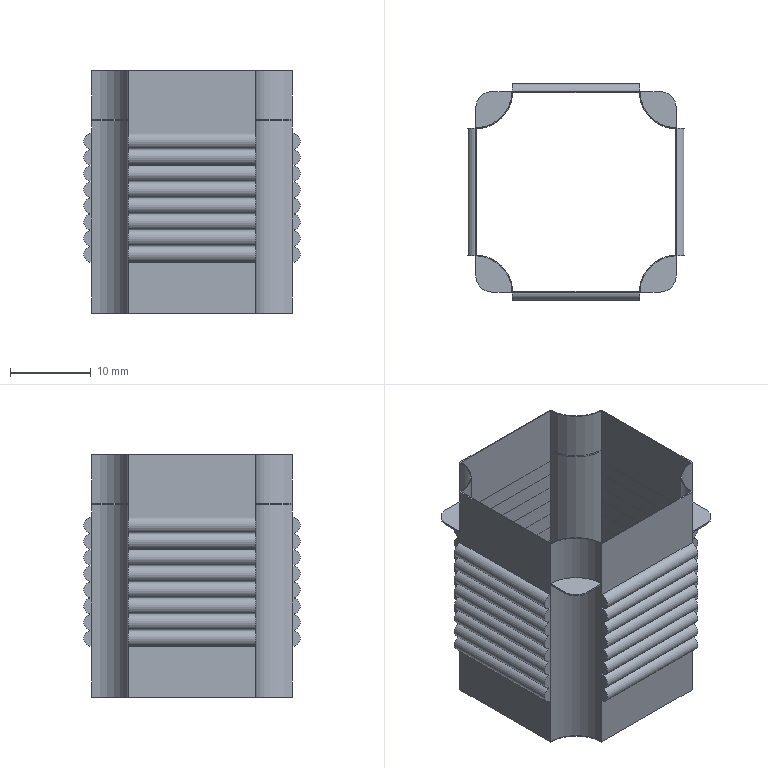Component | NX | STEPPER_MID | 1 solid | 134 faces | volume 1079 mm3 | plane 86 | cylinder 48 | commonest cylinder face diameters 2 x32 9.2 x8 9.4 x4 4 x4